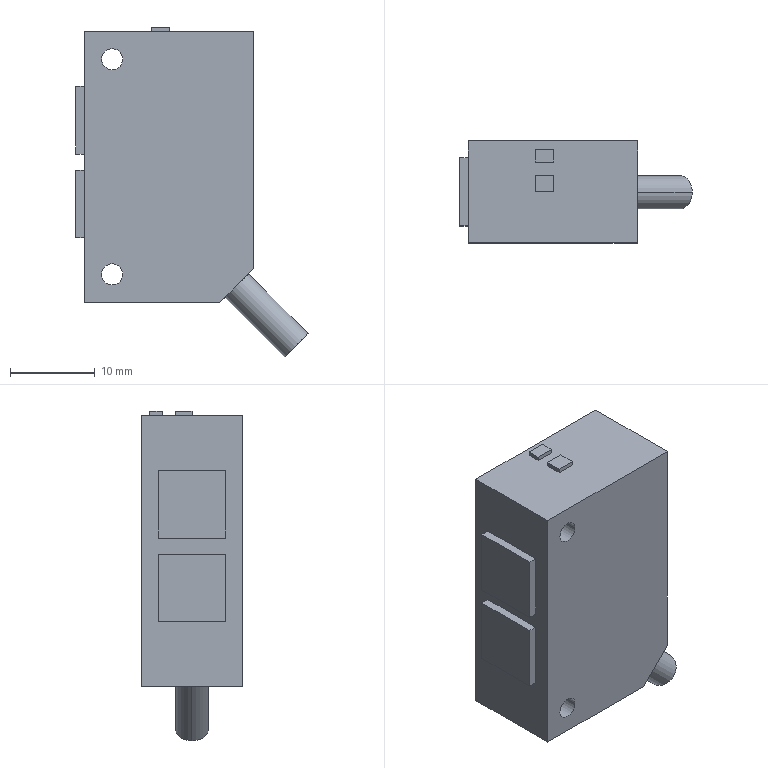Component | SolidWorks | Q20NRBanner-2 | 1 solid | 34 faces | box 27.45 x 12 x 38.95 mm | volume 7717 mm3 | plane 28 | cylinder 6 | commonest cylinder face diameters 2.5 x4 3.9 x2
build123d program:
from build123d import *

# Parameters (mm, degrees)
EXTRUDE1_DEPTH      = 6
EXTRUDE1_DEPTH_BACK = 6
SKETCH1_W           = 20
SKETCH1_H           = 32
M3_TAPPED_HOLE1_D   = 2.5
CHAMFER1_SIZE       = 4
SKETCH4_R           = 1.95
EXTRUDE2_DEPTH      = 10
SKETCH5_W           = 8
SKETCH5_H           = 8
EXTRUDE3_DEPTH      = 1
SKETCH12_W          = 2.2
SKETCH12_H          = 1.5
SKETCH12_H_2        = 1.92
EXTRUDE5_DEPTH      = 0.5


with BuildPart() as part:
    # Sketch1 → Extrude1 (new, two sides: drawn at the far end of the back side and taken through both)
    with BuildSketch(Plane.XY.offset(-EXTRUDE1_DEPTH_BACK)):
        with Locations((10, 16)):
            Rectangle(SKETCH1_W, SKETCH1_H)
    extrude(amount=EXTRUDE1_DEPTH + EXTRUDE1_DEPTH_BACK)

    # M3 Tapped Hole1 (through all)
    with Locations(Plane.XY.offset(6)):
        with Locations((3.3, 28.7), (3.3, 3.3)):
            Hole(M3_TAPPED_HOLE1_D / 2)

    # Chamfer1
    chamfer1_edges = [part.edges().sort_by_distance(p)[0] for p in [
        (20, 0, 0),
    ]]
    chamfer(chamfer1_edges, length=CHAMFER1_SIZE)

    # Sketch4 → Extrude2 (add)
    with BuildSketch(Plane(origin=(8, -8, 0), x_dir=(0, 0, -1), z_dir=(0.7071, -0.7071, 0))):
        with Locations(Location((0, 14.141, 0), (0, 0, 90))):
            Circle(SKETCH4_R)
    extrude(amount=EXTRUDE2_DEPTH)

    # Sketch5 → Extrude3 (add)
    with BuildSketch(Plane(origin=(0, 0, 0), x_dir=(0, 0, -1), z_dir=(1, 0, 0))):
        with Locations((0, 21.5)):
            Rectangle(SKETCH5_W, SKETCH5_H)
        with Locations((0, 11.6)):
            Rectangle(SKETCH5_W, SKETCH5_H)
    extrude(amount=-EXTRUDE3_DEPTH)

    # Sketch12 → Extrude5 (add)
    with BuildSketch(Plane(origin=(0, 32, 0), x_dir=(1, 0, 0), z_dir=(0, 1, 0))):
        with Locations((9, 4.25)):
            Rectangle(SKETCH12_W, SKETCH12_H)
        with Locations((9, 0.9598)):
            Rectangle(SKETCH12_W, SKETCH12_H_2)
    extrude(amount=EXTRUDE5_DEPTH)


solid = part.part

# Placed as in the assembly
solid = solid.moved(Location((-451.508, -99.092, 269.188), (90, 0, 0)))
STEP:
#1=CARTESIAN_POINT('',(-16.735,-3.901,10.453));
#2=VERTEX_POINT('',#1);
#3=CARTESIAN_POINT('',(-16.843,-3.901,10.344));
#4=VERTEX_POINT('',#3);
#5=CARTESIAN_POINT('',(-16.789,-3.901,10.398));
#6=DIRECTION('',(0.7071,0.,-0.7071));
#7=DIRECTION('',(0.7071,0.,0.7071));
#8=AXIS2_PLACEMENT_3D('',#5,#6,#7);
#9=CIRCLE('',#8,0.07677);
#10=EDGE_CURVE('',#2,#4,#9,.T.);
#11=ORIENTED_EDGE('',*,*,#10,.F.);
#12=CARTESIAN_POINT('',(-17.013,-3.901,10.731));
#13=VERTEX_POINT('',#12);
#14=CARTESIAN_POINT('',(-16.735,-3.901,10.453));
#15=DIRECTION('',(-0.7071,-0.,0.7071));
#16=VECTOR('',#15,39.37);
#17=LINE('',#14,#16);
#18=EDGE_CURVE('',#2,#13,#17,.T.);
#19=ORIENTED_EDGE('',*,*,#18,.T.);
#20=CARTESIAN_POINT('',(-17.122,-3.901,10.622));
#21=VERTEX_POINT('',#20);
#22=CARTESIAN_POINT('',(-17.067,-3.901,10.677));
#23=DIRECTION('',(0.7071,0.,-0.7071));
#24=DIRECTION('',(0.7071,0.,0.7071));
#25=AXIS2_PLACEMENT_3D('',#22,#23,#24);
#26=CIRCLE('',#25,0.07677);
#27=EDGE_CURVE('',#13,#21,#26,.T.);
#28=ORIENTED_EDGE('',*,*,#27,.T.);
#29=CARTESIAN_POINT('',(-16.843,-3.901,10.344));
#30=DIRECTION('',(-0.7071,-0.,0.7071));
#31=VECTOR('',#30,39.37);
#32=LINE('',#29,#31);
#33=EDGE_CURVE('',#4,#21,#32,.T.);
#34=ORIENTED_EDGE('',*,*,#33,.F.);
#35=EDGE_LOOP('',(#11,#19,#28,#34));
#36=FACE_OUTER_BOUND('',#35,.T.);
#37=CARTESIAN_POINT('',(-16.789,-3.901,10.398));
#38=DIRECTION('',(-0.7071,-0.,0.7071));
#39=DIRECTION('',(-0.7071,-0.,-0.7071));
#40=AXIS2_PLACEMENT_3D('',#37,#38,#39);
#41=CYLINDRICAL_SURFACE('',#40,0.07677);
#42=ADVANCED_FACE('',(#36),#41,.T.);
#43=CARTESIAN_POINT('',(-17.695,-3.665,11.728));
#44=VERTEX_POINT('',#43);
#45=CARTESIAN_POINT('',(-17.597,-3.665,11.728));
#46=VERTEX_POINT('',#45);
#47=CARTESIAN_POINT('',(-17.646,-3.665,11.728));
#48=DIRECTION('',(0.,-1.,0.));
#49=DIRECTION('',(1.,0.,0.));
#50=AXIS2_PLACEMENT_3D('',#47,#48,#49);
#51=CIRCLE('',#50,0.04921);
#52=EDGE_CURVE('',#44,#46,#51,.T.);
#53=ORIENTED_EDGE('',*,*,#52,.F.);
#54=CARTESIAN_POINT('',(-17.695,-4.137,11.728));
#55=VERTEX_POINT('',#54);
#56=CARTESIAN_POINT('',(-17.695,-4.137,11.728));
#57=DIRECTION('',(0.,-1.,0.));
#58=VECTOR('',#57,39.37);
#59=LINE('',#56,#58);
#60=EDGE_CURVE('',#44,#55,#59,.T.);
#61=ORIENTED_EDGE('',*,*,#60,.T.);
#62=CARTESIAN_POINT('',(-17.597,-4.137,11.728));
#63=VERTEX_POINT('',#62);
#64=CARTESIAN_POINT('',(-17.646,-4.137,11.728));
#65=DIRECTION('',(0.,-1.,0.));
#66=DIRECTION('',(1.,0.,0.));
#67=AXIS2_PLACEMENT_3D('',#64,#65,#66);
#68=CIRCLE('',#67,0.04921);
#69=EDGE_CURVE('',#55,#63,#68,.T.);
#70=ORIENTED_EDGE('',*,*,#69,.T.);
#71=CARTESIAN_POINT('',(-17.597,-4.137,11.728));
#72=DIRECTION('',(0.,-1.,0.));
#73=VECTOR('',#72,39.37);
#74=LINE('',#71,#73);
#75=EDGE_CURVE('',#46,#63,#74,.T.);
#76=ORIENTED_EDGE('',*,*,#75,.F.);
#77=EDGE_LOOP('',(#53,#61,#70,#76));
#78=FACE_OUTER_BOUND('',#77,.T.);
#79=CARTESIAN_POINT('',(-17.646,-4.137,11.728));
#80=DIRECTION('',(0.,-1.,0.));
#81=DIRECTION('',(1.,0.,0.));
#82=AXIS2_PLACEMENT_3D('',#79,#80,#81);
#83=CYLINDRICAL_SURFACE('',#82,0.04921);
#84=ADVANCED_FACE('',(#78),#83,.F.);
#85=CARTESIAN_POINT('',(-17.695,-3.665,10.728));
#86=VERTEX_POINT('',#85);
#87=CARTESIAN_POINT('',(-17.597,-3.665,10.728));
#88=VERTEX_POINT('',#87);
#89=CARTESIAN_POINT('',(-17.646,-3.665,10.728));
#90=DIRECTION('',(0.,-1.,0.));
#91=DIRECTION('',(1.,0.,0.));
#92=AXIS2_PLACEMENT_3D('',#89,#90,#91);
#93=CIRCLE('',#92,0.04921);
#94=EDGE_CURVE('',#86,#88,#93,.T.);
#95=ORIENTED_EDGE('',*,*,#94,.F.);
#96=CARTESIAN_POINT('',(-17.695,-4.137,10.728));
#97=VERTEX_POINT('',#96);
#98=CARTESIAN_POINT('',(-17.695,-4.137,10.728));
#99=DIRECTION('',(0.,-1.,0.));
#100=VECTOR('',#99,39.37);
#101=LINE('',#98,#100);
#102=EDGE_CURVE('',#86,#97,#101,.T.);
#103=ORIENTED_EDGE('',*,*,#102,.T.);
#104=CARTESIAN_POINT('',(-17.597,-4.137,10.728));
#105=VERTEX_POINT('',#104);
#106=CARTESIAN_POINT('',(-17.646,-4.137,10.728));
#107=DIRECTION('',(0.,-1.,0.));
#108=DIRECTION('',(1.,0.,0.));
#109=AXIS2_PLACEMENT_3D('',#106,#107,#108);
#110=CIRCLE('',#109,0.04921);
#111=EDGE_CURVE('',#97,#105,#110,.T.);
#112=ORIENTED_EDGE('',*,*,#111,.T.);
#113=CARTESIAN_POINT('',(-17.597,-4.137,10.728));
#114=DIRECTION('',(0.,-1.,0.));
#115=VECTOR('',#114,39.37);
#116=LINE('',#113,#115);
#117=EDGE_CURVE('',#88,#105,#116,.T.);
#118=ORIENTED_EDGE('',*,*,#117,.F.);
#119=EDGE_LOOP('',(#95,#103,#112,#118));
#120=FACE_OUTER_BOUND('',#119,.T.);
#121=CARTESIAN_POINT('',(-17.646,-4.137,10.728));
#122=DIRECTION('',(0.,-1.,0.));
#123=DIRECTION('',(1.,0.,0.));
#124=AXIS2_PLACEMENT_3D('',#121,#122,#123);
#125=CYLINDRICAL_SURFACE('',#124,0.04921);
#126=ADVANCED_FACE('',(#120),#125,.F.);
#127=CARTESIAN_POINT('',(-17.465,-3.763,11.858));
#128=VERTEX_POINT('',#127);
#129=CARTESIAN_POINT('',(-17.378,-3.763,11.858));
#130=VERTEX_POINT('',#129);
#131=CARTESIAN_POINT('',(-17.465,-3.763,11.858));
#132=DIRECTION('',(1.,0.,-0.));
#133=VECTOR('',#132,39.37);
#134=LINE('',#131,#133);
#135=EDGE_CURVE('',#128,#130,#134,.T.);
#136=ORIENTED_EDGE('',*,*,#135,.F.);
#137=CARTESIAN_POINT('',(-17.465,-3.704,11.858));
#138=VERTEX_POINT('',#137);
#139=CARTESIAN_POINT('',(-17.465,-3.704,11.858));
#140=DIRECTION('',(0.,-1.,0.));
#141=VECTOR('',#140,39.37);
#142=LINE('',#139,#141);
#143=EDGE_CURVE('',#138,#128,#142,.T.);
#144=ORIENTED_EDGE('',*,*,#143,.F.);
#145=CARTESIAN_POINT('',(-17.378,-3.704,11.858));
#146=VERTEX_POINT('',#145);
#147=CARTESIAN_POINT('',(-17.465,-3.704,11.858));
#148=DIRECTION('',(-1.,-0.,0.));
#149=VECTOR('',#148,39.37);
#150=LINE('',#147,#149);
#151=EDGE_CURVE('',#146,#138,#150,.T.);
#152=ORIENTED_EDGE('',*,*,#151,.F.);
#153=CARTESIAN_POINT('',(-17.378,-3.704,11.858));
#154=DIRECTION('',(-0.,1.,-0.));
#155=VECTOR('',#154,39.37);
#156=LINE('',#153,#155);
#157=EDGE_CURVE('',#130,#146,#156,.T.);
#158=ORIENTED_EDGE('',*,*,#157,.F.);
#159=EDGE_LOOP('',(#136,#144,#152,#158));
#160=FACE_BOUND('',#159,.T.);
#161=CARTESIAN_POINT('',(-17.776,-3.665,11.858));
#162=VERTEX_POINT('',#161);
#163=CARTESIAN_POINT('',(-17.776,-4.137,11.858));
#164=VERTEX_POINT('',#163);
#165=CARTESIAN_POINT('',(-17.776,-3.665,11.858));
#166=DIRECTION('',(0.,-1.,0.));
#167=VECTOR('',#166,39.37);
#168=LINE('',#165,#167);
#169=EDGE_CURVE('',#162,#164,#168,.T.);
#170=ORIENTED_EDGE('',*,*,#169,.T.);
#171=CARTESIAN_POINT('',(-16.988,-4.137,11.858));
#172=VERTEX_POINT('',#171);
#173=CARTESIAN_POINT('',(-17.776,-4.137,11.858));
#174=DIRECTION('',(-1.,-0.,0.));
#175=VECTOR('',#174,39.37);
#176=LINE('',#173,#175);
#177=EDGE_CURVE('',#172,#164,#176,.T.);
#178=ORIENTED_EDGE('',*,*,#177,.F.);
#179=CARTESIAN_POINT('',(-16.988,-3.665,11.858));
#180=VERTEX_POINT('',#179);
#181=CARTESIAN_POINT('',(-16.988,-3.665,11.858));
#182=DIRECTION('',(0.,-1.,0.));
#183=VECTOR('',#182,39.37);
#184=LINE('',#181,#183);
#185=EDGE_CURVE('',#180,#172,#184,.T.);
#186=ORIENTED_EDGE('',*,*,#185,.F.);
#187=CARTESIAN_POINT('',(-17.776,-3.665,11.858));
#188=DIRECTION('',(-1.,-0.,0.));
#189=VECTOR('',#188,39.37);
#190=LINE('',#187,#189);
#191=EDGE_CURVE('',#180,#162,#190,.T.);
#192=ORIENTED_EDGE('',*,*,#191,.T.);
#193=EDGE_LOOP('',(#170,#178,#186,#192));
#194=FACE_OUTER_BOUND('',#193,.T.);
#195=CARTESIAN_POINT('',(-17.465,-3.901,11.858));
#196=VERTEX_POINT('',#195);
#197=CARTESIAN_POINT('',(-17.378,-3.901,11.858));
#198=VERTEX_POINT('',#197);
#199=CARTESIAN_POINT('',(-17.465,-3.901,11.858));
#200=DIRECTION('',(1.,0.,-0.));
#201=VECTOR('',#200,39.37);
#202=LINE('',#199,#201);
#203=EDGE_CURVE('',#196,#198,#202,.T.);
#204=ORIENTED_EDGE('',*,*,#203,.F.);
#205=CARTESIAN_POINT('',(-17.465,-3.826,11.858));
#206=VERTEX_POINT('',#205);
#207=CARTESIAN_POINT('',(-17.465,-3.826,11.858));
#208=DIRECTION('',(0.,-1.,0.));
#209=VECTOR('',#208,39.37);
#210=LINE('',#207,#209);
#211=EDGE_CURVE('',#206,#196,#210,.T.);
#212=ORIENTED_EDGE('',*,*,#211,.F.);
#213=CARTESIAN_POINT('',(-17.378,-3.826,11.858));
#214=VERTEX_POINT('',#213);
#215=CARTESIAN_POINT('',(-17.465,-3.826,11.858));
#216=DIRECTION('',(-1.,-0.,0.));
#217=VECTOR('',#216,39.37);
#218=LINE('',#215,#217);
#219=EDGE_CURVE('',#214,#206,#218,.T.);
#220=ORIENTED_EDGE('',*,*,#219,.F.);
#221=CARTESIAN_POINT('',(-17.378,-3.826,11.858));
#222=DIRECTION('',(-0.,1.,-0.));
#223=VECTOR('',#222,39.37);
#224=LINE('',#221,#223);
#225=EDGE_CURVE('',#198,#214,#224,.T.);
#226=ORIENTED_EDGE('',*,*,#225,.F.);
#227=EDGE_LOOP('',(#204,#212,#220,#226));
#228=FACE_BOUND('',#227,.T.);
#229=CARTESIAN_POINT('',(-17.776,-3.665,11.858));
#230=DIRECTION('',(0.,0.,1.));
#231=DIRECTION('',(0.,-1.,0.));
#232=AXIS2_PLACEMENT_3D('',#229,#230,#231);
#233=PLANE('',#232);
#234=ADVANCED_FACE('',(#160,#194,#228),#233,.T.);
#235=CARTESIAN_POINT('',(-16.988,-3.665,10.755));
#236=VERTEX_POINT('',#235);
#237=CARTESIAN_POINT('',(-17.146,-3.665,10.598));
#238=VERTEX_POINT('',#237);
#239=CARTESIAN_POINT('',(-16.831,-3.665,10.913));
#240=DIRECTION('',(-0.7071,-0.,-0.7071));
#241=VECTOR('',#240,39.37);
#242=LINE('',#239,#241);
#243=EDGE_CURVE('',#236,#238,#242,.T.);
#244=ORIENTED_EDGE('',*,*,#243,.F.);
#245=CARTESIAN_POINT('',(-16.988,-4.137,10.755));
#246=VERTEX_POINT('',#245);
#247=CARTESIAN_POINT('',(-16.988,-3.665,10.755));
#248=DIRECTION('',(-0.,1.,-0.));
#249=VECTOR('',#248,39.37);
#250=LINE('',#247,#249);
#251=EDGE_CURVE('',#246,#236,#250,.T.);
#252=ORIENTED_EDGE('',*,*,#251,.F.);
#253=CARTESIAN_POINT('',(-17.146,-4.137,10.598));
#254=VERTEX_POINT('',#253);
#255=CARTESIAN_POINT('',(-17.146,-4.137,10.598));
#256=DIRECTION('',(0.7071,0.,0.7071));
#257=VECTOR('',#256,39.37);
#258=LINE('',#255,#257);
#259=EDGE_CURVE('',#254,#246,#258,.T.);
#260=ORIENTED_EDGE('',*,*,#259,.F.);
#261=CARTESIAN_POINT('',(-17.146,-3.665,10.598));
#262=DIRECTION('',(0.,-1.,0.));
#263=VECTOR('',#262,39.37);
#264=LINE('',#261,#263);
#265=EDGE_CURVE('',#238,#254,#264,.T.);
#266=ORIENTED_EDGE('',*,*,#265,.F.);
#267=EDGE_LOOP('',(#244,#252,#260,#266));
#268=FACE_OUTER_BOUND('',#267,.T.);
#269=CARTESIAN_POINT('',(-17.067,-3.901,10.677));
#270=DIRECTION('',(0.7071,0.,-0.7071));
#271=DIRECTION('',(0.7071,0.,0.7071));
#272=AXIS2_PLACEMENT_3D('',#269,#270,#271);
#273=CIRCLE('',#272,0.07677);
#274=EDGE_CURVE('',#21,#13,#273,.T.);
#275=ORIENTED_EDGE('',*,*,#274,.F.);
#276=ORIENTED_EDGE('',*,*,#27,.F.);
#277=EDGE_LOOP('',(#275,#276));
#278=FACE_BOUND('',#277,.T.);
#279=CARTESIAN_POINT('',(-17.146,-3.665,10.598));
#280=DIRECTION('',(-0.7071,-0.,0.7071));
#281=DIRECTION('',(-0.7071,-0.,-0.7071));
#282=AXIS2_PLACEMENT_3D('',#279,#280,#281);
#283=PLANE('',#282);
#284=ADVANCED_FACE('',(#268,#278),#283,.F.);
#285=CARTESIAN_POINT('',(-17.776,-4.059,11.212));
#286=VERTEX_POINT('',#285);
#287=CARTESIAN_POINT('',(-17.776,-4.059,10.897));
#288=VERTEX_POINT('',#287);
#289=CARTESIAN_POINT('',(-17.776,-4.059,11.212));
#290=DIRECTION('',(-0.,0.,-1.));
#291=VECTOR('',#290,39.37);
#292=LINE('',#289,#291);
#293=EDGE_CURVE('',#286,#288,#292,.T.);
#294=ORIENTED_EDGE('',*,*,#293,.T.);
#295=CARTESIAN_POINT('',(-17.776,-3.744,10.897));
#296=VERTEX_POINT('',#295);
#297=CARTESIAN_POINT('',(-17.776,-4.059,10.897));
#298=DIRECTION('',(-0.,1.,-0.));
#299=VECTOR('',#298,39.37);
#300=LINE('',#297,#299);
#301=EDGE_CURVE('',#288,#296,#300,.T.);
#302=ORIENTED_EDGE('',*,*,#301,.T.);
#303=CARTESIAN_POINT('',(-17.776,-3.744,11.212));
#304=VERTEX_POINT('',#303);
#305=CARTESIAN_POINT('',(-17.776,-3.744,11.212));
#306=DIRECTION('',(0.,-0.,1.));
#307=VECTOR('',#306,39.37);
#308=LINE('',#305,#307);
#309=EDGE_CURVE('',#296,#304,#308,.T.);
#310=ORIENTED_EDGE('',*,*,#309,.T.);
#311=CARTESIAN_POINT('',(-17.776,-4.059,11.212));
#312=DIRECTION('',(0.,-1.,-0.));
#313=VECTOR('',#312,39.37);
#314=LINE('',#311,#313);
#315=EDGE_CURVE('',#304,#286,#314,.T.);
#316=ORIENTED_EDGE('',*,*,#315,.T.);
#317=EDGE_LOOP('',(#294,#302,#310,#316));
#318=FACE_BOUND('',#317,.T.);
#319=CARTESIAN_POINT('',(-17.776,-4.059,11.602));
#320=VERTEX_POINT('',#319);
#321=CARTESIAN_POINT('',(-17.776,-4.059,11.287));
#322=VERTEX_POINT('',#321);
#323=CARTESIAN_POINT('',(-17.776,-4.059,11.602));
#324=DIRECTION('',(-0.,-0.,-1.));
#325=VECTOR('',#324,39.37);
#326=LINE('',#323,#325);
#327=EDGE_CURVE('',#320,#322,#326,.T.);
#328=ORIENTED_EDGE('',*,*,#327,.T.);
#329=CARTESIAN_POINT('',(-17.776,-3.744,11.287));
#330=VERTEX_POINT('',#329);
#331=CARTESIAN_POINT('',(-17.776,-4.059,11.287));
#332=DIRECTION('',(-0.,1.,-0.));
#333=VECTOR('',#332,39.37);
#334=LINE('',#331,#333);
#335=EDGE_CURVE('',#322,#330,#334,.T.);
#336=ORIENTED_EDGE('',*,*,#335,.T.);
#337=CARTESIAN_POINT('',(-17.776,-3.744,11.602));
#338=VERTEX_POINT('',#337);
#339=CARTESIAN_POINT('',(-17.776,-3.744,11.602));
#340=DIRECTION('',(0.,0.,1.));
#341=VECTOR('',#340,39.37);
#342=LINE('',#339,#341);
#343=EDGE_CURVE('',#330,#338,#342,.T.);
#344=ORIENTED_EDGE('',*,*,#343,.T.);
#345=CARTESIAN_POINT('',(-17.776,-4.059,11.602));
#346=DIRECTION('',(0.,-1.,0.));
#347=VECTOR('',#346,39.37);
#348=LINE('',#345,#347);
#349=EDGE_CURVE('',#338,#320,#348,.T.);
#350=ORIENTED_EDGE('',*,*,#349,.T.);
#351=EDGE_LOOP('',(#328,#336,#344,#350));
#352=FACE_BOUND('',#351,.T.);
#353=CARTESIAN_POINT('',(-17.776,-3.665,10.598));
#354=VERTEX_POINT('',#353);
#355=CARTESIAN_POINT('',(-17.776,-4.137,10.598));
#356=VERTEX_POINT('',#355);
#357=CARTESIAN_POINT('',(-17.776,-3.665,10.598));
#358=DIRECTION('',(0.,-1.,0.));
#359=VECTOR('',#358,39.37);
#360=LINE('',#357,#359);
#361=EDGE_CURVE('',#354,#356,#360,.T.);
#362=ORIENTED_EDGE('',*,*,#361,.T.);
#363=CARTESIAN_POINT('',(-17.776,-4.137,10.598));
#364=DIRECTION('',(-0.,-0.,-1.));
#365=VECTOR('',#364,39.37);
#366=LINE('',#363,#365);
#367=EDGE_CURVE('',#164,#356,#366,.T.);
#368=ORIENTED_EDGE('',*,*,#367,.F.);
#369=ORIENTED_EDGE('',*,*,#169,.F.);
#370=CARTESIAN_POINT('',(-17.776,-3.665,10.598));
#371=DIRECTION('',(-0.,-0.,-1.));
#372=VECTOR('',#371,39.37);
#373=LINE('',#370,#372);
#374=EDGE_CURVE('',#162,#354,#373,.T.);
#375=ORIENTED_EDGE('',*,*,#374,.T.);
#376=EDGE_LOOP('',(#362,#368,#369,#375));
#377=FACE_OUTER_BOUND('',#376,.T.);
#378=CARTESIAN_POINT('',(-17.776,-3.665,10.598));
#379=DIRECTION('',(-1.,-0.,0.));
#380=DIRECTION('',(0.,-1.,0.));
#381=AXIS2_PLACEMENT_3D('',#378,#379,#380);
#382=PLANE('',#381);
#383=ADVANCED_FACE('',(#318,#352,#377),#382,.T.);
#384=CARTESIAN_POINT('',(-16.988,-4.137,10.598));
#385=DIRECTION('',(0.,0.,1.));
#386=VECTOR('',#385,39.37);
#387=LINE('',#384,#386);
#388=EDGE_CURVE('',#246,#172,#387,.T.);
#389=ORIENTED_EDGE('',*,*,#388,.F.);
#390=ORIENTED_EDGE('',*,*,#251,.T.);
#391=CARTESIAN_POINT('',(-16.988,-3.665,10.598));
#392=DIRECTION('',(0.,0.,1.));
#393=VECTOR('',#392,39.37);
#394=LINE('',#391,#393);
#395=EDGE_CURVE('',#236,#180,#394,.T.);
#396=ORIENTED_EDGE('',*,*,#395,.T.);
#397=ORIENTED_EDGE('',*,*,#185,.T.);
#398=EDGE_LOOP('',(#389,#390,#396,#397));
#399=FACE_OUTER_BOUND('',#398,.T.);
#400=CARTESIAN_POINT('',(-16.988,-3.665,10.598));
#401=DIRECTION('',(1.,0.,-0.));
#402=DIRECTION('',(-0.,1.,-0.));
#403=AXIS2_PLACEMENT_3D('',#400,#401,#402);
#404=PLANE('',#403);
#405=ADVANCED_FACE('',(#399),#404,.T.);
#406=CARTESIAN_POINT('',(-17.776,-3.665,10.598));
#407=DIRECTION('',(1.,0.,-0.));
#408=VECTOR('',#407,39.37);
#409=LINE('',#406,#408);
#410=EDGE_CURVE('',#354,#238,#409,.T.);
#411=ORIENTED_EDGE('',*,*,#410,.T.);
#412=ORIENTED_EDGE('',*,*,#265,.T.);
#413=CARTESIAN_POINT('',(-17.776,-4.137,10.598));
#414=DIRECTION('',(1.,0.,-0.));
#415=VECTOR('',#414,39.37);
#416=LINE('',#413,#415);
#417=EDGE_CURVE('',#356,#254,#416,.T.);
#418=ORIENTED_EDGE('',*,*,#417,.F.);
#419=ORIENTED_EDGE('',*,*,#361,.F.);
#420=EDGE_LOOP('',(#411,#412,#418,#419));
#421=FACE_OUTER_BOUND('',#420,.T.);
#422=CARTESIAN_POINT('',(-17.776,-3.665,10.598));
#423=DIRECTION('',(-0.,-0.,-1.));
#424=DIRECTION('',(-0.,1.,-0.));
#425=AXIS2_PLACEMENT_3D('',#422,#423,#424);
#426=PLANE('',#425);
#427=ADVANCED_FACE('',(#421),#426,.T.);
#428=CARTESIAN_POINT('',(-17.646,-3.665,11.728));
#429=DIRECTION('',(0.,-1.,0.));
#430=DIRECTION('',(1.,0.,0.));
#431=AXIS2_PLACEMENT_3D('',#428,#429,#430);
#432=CIRCLE('',#431,0.04921);
#433=EDGE_CURVE('',#46,#44,#432,.T.);
#434=ORIENTED_EDGE('',*,*,#433,.T.);
#435=ORIENTED_EDGE('',*,*,#52,.T.);
#436=EDGE_LOOP('',(#434,#435));
#437=FACE_BOUND('',#436,.T.);
#438=CARTESIAN_POINT('',(-17.646,-3.665,10.728));
#439=DIRECTION('',(0.,-1.,0.));
#440=DIRECTION('',(1.,0.,0.));
#441=AXIS2_PLACEMENT_3D('',#438,#439,#440);
#442=CIRCLE('',#441,0.04921);
#443=EDGE_CURVE('',#88,#86,#442,.T.);
#444=ORIENTED_EDGE('',*,*,#443,.T.);
#445=ORIENTED_EDGE('',*,*,#94,.T.);
#446=EDGE_LOOP('',(#444,#445));
#447=FACE_BOUND('',#446,.T.);
#448=ORIENTED_EDGE('',*,*,#395,.F.);
#449=ORIENTED_EDGE('',*,*,#243,.T.);
#450=ORIENTED_EDGE('',*,*,#410,.F.);
#451=ORIENTED_EDGE('',*,*,#374,.F.);
#452=ORIENTED_EDGE('',*,*,#191,.F.);
#453=EDGE_LOOP('',(#448,#449,#450,#451,#452));
#454=FACE_OUTER_BOUND('',#453,.T.);
#455=CARTESIAN_POINT('',(-17.776,-3.665,11.858));
#456=DIRECTION('',(-0.,1.,-0.));
#457=DIRECTION('',(-1.,-0.,0.));
#458=AXIS2_PLACEMENT_3D('',#455,#456,#457);
#459=PLANE('',#458);
#460=ADVANCED_FACE('',(#437,#447,#454),#459,.T.);
#461=CARTESIAN_POINT('',(-17.646,-4.137,11.728));
#462=DIRECTION('',(0.,-1.,0.));
#463=DIRECTION('',(1.,0.,0.));
#464=AXIS2_PLACEMENT_3D('',#461,#462,#463);
#465=CIRCLE('',#464,0.04921);
#466=EDGE_CURVE('',#63,#55,#465,.T.);
#467=ORIENTED_EDGE('',*,*,#466,.F.);
#468=ORIENTED_EDGE('',*,*,#69,.F.);
#469=EDGE_LOOP('',(#467,#468));
#470=FACE_BOUND('',#469,.T.);
#471=CARTESIAN_POINT('',(-17.646,-4.137,10.728));
#472=DIRECTION('',(0.,-1.,0.));
#473=DIRECTION('',(1.,0.,0.));
#474=AXIS2_PLACEMENT_3D('',#471,#472,#473);
#475=CIRCLE('',#474,0.04921);
#476=EDGE_CURVE('',#105,#97,#475,.T.);
#477=ORIENTED_EDGE('',*,*,#476,.F.);
#478=ORIENTED_EDGE('',*,*,#111,.F.);
#479=EDGE_LOOP('',(#477,#478));
#480=FACE_BOUND('',#479,.T.);
#481=ORIENTED_EDGE('',*,*,#417,.T.);
#482=ORIENTED_EDGE('',*,*,#259,.T.);
#483=ORIENTED_EDGE('',*,*,#388,.T.);
#484=ORIENTED_EDGE('',*,*,#177,.T.);
#485=ORIENTED_EDGE('',*,*,#367,.T.);
#486=EDGE_LOOP('',(#481,#482,#483,#484,#485));
#487=FACE_OUTER_BOUND('',#486,.T.);
#488=CARTESIAN_POINT('',(-17.776,-4.137,11.858));
#489=DIRECTION('',(-0.,1.,-0.));
#490=DIRECTION('',(-1.,-0.,0.));
#491=AXIS2_PLACEMENT_3D('',#488,#489,#490);
#492=PLANE('',#491);
#493=ADVANCED_FACE('',(#470,#480,#487),#492,.F.);
#494=ORIENTED_EDGE('',*,*,#102,.F.);
#495=ORIENTED_EDGE('',*,*,#443,.F.);
#496=ORIENTED_EDGE('',*,*,#117,.T.);
#497=ORIENTED_EDGE('',*,*,#476,.T.);
#498=EDGE_LOOP('',(#494,#495,#496,#497));
#499=FACE_OUTER_BOUND('',#498,.T.);
#500=CARTESIAN_POINT('',(-17.646,-4.137,10.728));
#501=DIRECTION('',(0.,-1.,0.));
#502=DIRECTION('',(1.,0.,0.));
#503=AXIS2_PLACEMENT_3D('',#500,#501,#502);
#504=CYLINDRICAL_SURFACE('',#503,0.04921);
#505=ADVANCED_FACE('',(#499),#504,.F.);
#506=ORIENTED_EDGE('',*,*,#60,.F.);
#507=ORIENTED_EDGE('',*,*,#433,.F.);
#508=ORIENTED_EDGE('',*,*,#75,.T.);
#509=ORIENTED_EDGE('',*,*,#466,.T.);
#510=EDGE_LOOP('',(#506,#507,#508,#509));
#511=FACE_OUTER_BOUND('',#510,.T.);
#512=CARTESIAN_POINT('',(-17.646,-4.137,11.728));
#513=DIRECTION('',(0.,-1.,0.));
#514=DIRECTION('',(1.,0.,0.));
#515=AXIS2_PLACEMENT_3D('',#512,#513,#514);
#516=CYLINDRICAL_SURFACE('',#515,0.04921);
#517=ADVANCED_FACE('',(#511),#516,.F.);
#518=ORIENTED_EDGE('',*,*,#18,.F.);
#519=CARTESIAN_POINT('',(-16.789,-3.901,10.398));
#520=DIRECTION('',(0.7071,0.,-0.7071));
#521=DIRECTION('',(0.7071,0.,0.7071));
#522=AXIS2_PLACEMENT_3D('',#519,#520,#521);
#523=CIRCLE('',#522,0.07677);
#524=EDGE_CURVE('',#4,#2,#523,.T.);
#525=ORIENTED_EDGE('',*,*,#524,.F.);
#526=ORIENTED_EDGE('',*,*,#33,.T.);
#527=ORIENTED_EDGE('',*,*,#274,.T.);
#528=EDGE_LOOP('',(#518,#525,#526,#527));
#529=FACE_OUTER_BOUND('',#528,.T.);
#530=CARTESIAN_POINT('',(-16.789,-3.901,10.398));
#531=DIRECTION('',(-0.7071,-0.,0.7071));
#532=DIRECTION('',(-0.7071,-0.,-0.7071));
#533=AXIS2_PLACEMENT_3D('',#530,#531,#532);
#534=CYLINDRICAL_SURFACE('',#533,0.07677);
#535=ADVANCED_FACE('',(#529),#534,.T.);
#536=ORIENTED_EDGE('',*,*,#524,.T.);
#537=ORIENTED_EDGE('',*,*,#10,.T.);
#538=EDGE_LOOP('',(#536,#537));
#539=FACE_OUTER_BOUND('',#538,.T.);
#540=CARTESIAN_POINT('',(-16.789,-3.901,10.398));
#541=DIRECTION('',(0.7071,0.,-0.7071));
#542=DIRECTION('',(0.7071,0.,0.7071));
#543=AXIS2_PLACEMENT_3D('',#540,#541,#542);
#544=PLANE('',#543);
#545=ADVANCED_FACE('',(#539),#544,.T.);
#546=ORIENTED_EDGE('',*,*,#327,.F.);
#547=CARTESIAN_POINT('',(-17.815,-4.059,11.602));
#548=VERTEX_POINT('',#547);
#549=CARTESIAN_POINT('',(-17.815,-4.059,11.602));
#550=DIRECTION('',(1.,0.,-0.));
#551=VECTOR('',#550,39.37);
#552=LINE('',#549,#551);
#553=EDGE_CURVE('',#548,#320,#552,.T.);
#554=ORIENTED_EDGE('',*,*,#553,.F.);
#555=CARTESIAN_POINT('',(-17.815,-4.059,11.287));
#556=VERTEX_POINT('',#555);
#557=CARTESIAN_POINT('',(-17.815,-4.059,11.602));
#558=DIRECTION('',(-0.,-0.,-1.));
#559=VECTOR('',#558,39.37);
#560=LINE('',#557,#559);
#561=EDGE_CURVE('',#548,#556,#560,.T.);
#562=ORIENTED_EDGE('',*,*,#561,.T.);
#563=CARTESIAN_POINT('',(-17.815,-4.059,11.287));
#564=DIRECTION('',(1.,0.,-0.));
#565=VECTOR('',#564,39.37);
#566=LINE('',#563,#565);
#567=EDGE_CURVE('',#556,#322,#566,.T.);
#568=ORIENTED_EDGE('',*,*,#567,.T.);
#569=EDGE_LOOP('',(#546,#554,#562,#568));
#570=FACE_OUTER_BOUND('',#569,.T.);
#571=CARTESIAN_POINT('',(-17.815,-4.059,11.602));
#572=DIRECTION('',(0.,-1.,0.));
#573=DIRECTION('',(1.,0.,-0.));
#574=AXIS2_PLACEMENT_3D('',#571,#572,#573);
#575=PLANE('',#574);
#576=ADVANCED_FACE('',(#570),#575,.T.);
#577=ORIENTED_EDGE('',*,*,#349,.F.);
#578=CARTESIAN_POINT('',(-17.815,-3.744,11.602));
#579=VERTEX_POINT('',#578);
#580=CARTESIAN_POINT('',(-17.815,-3.744,11.602));
#581=DIRECTION('',(1.,0.,-0.));
#582=VECTOR('',#581,39.37);
#583=LINE('',#580,#582);
#584=EDGE_CURVE('',#579,#338,#583,.T.);
#585=ORIENTED_EDGE('',*,*,#584,.F.);
#586=CARTESIAN_POINT('',(-17.815,-4.059,11.602));
#587=DIRECTION('',(0.,-1.,0.));
#588=VECTOR('',#587,39.37);
#589=LINE('',#586,#588);
#590=EDGE_CURVE('',#579,#548,#589,.T.);
#591=ORIENTED_EDGE('',*,*,#590,.T.);
#592=ORIENTED_EDGE('',*,*,#553,.T.);
#593=EDGE_LOOP('',(#577,#585,#591,#592));
#594=FACE_OUTER_BOUND('',#593,.T.);
#595=CARTESIAN_POINT('',(-17.815,-4.059,11.602));
#596=DIRECTION('',(0.,0.,1.));
#597=DIRECTION('',(0.,-1.,0.));
#598=AXIS2_PLACEMENT_3D('',#595,#596,#597);
#599=PLANE('',#598);
#600=ADVANCED_FACE('',(#594),#599,.T.);
#601=ORIENTED_EDGE('',*,*,#343,.F.);
#602=CARTESIAN_POINT('',(-17.815,-3.744,11.287));
#603=VERTEX_POINT('',#602);
#604=CARTESIAN_POINT('',(-17.815,-3.744,11.287));
#605=DIRECTION('',(1.,0.,-0.));
#606=VECTOR('',#605,39.37);
#607=LINE('',#604,#606);
#608=EDGE_CURVE('',#603,#330,#607,.T.);
#609=ORIENTED_EDGE('',*,*,#608,.F.);
#610=CARTESIAN_POINT('',(-17.815,-3.744,11.602));
#611=DIRECTION('',(0.,0.,1.));
#612=VECTOR('',#611,39.37);
#613=LINE('',#610,#612);
#614=EDGE_CURVE('',#603,#579,#613,.T.);
#615=ORIENTED_EDGE('',*,*,#614,.T.);
#616=ORIENTED_EDGE('',*,*,#584,.T.);
#617=EDGE_LOOP('',(#601,#609,#615,#616));
#618=FACE_OUTER_BOUND('',#617,.T.);
#619=CARTESIAN_POINT('',(-17.815,-3.744,11.602));
#620=DIRECTION('',(-0.,1.,-0.));
#621=DIRECTION('',(-1.,-0.,0.));
#622=AXIS2_PLACEMENT_3D('',#619,#620,#621);
#623=PLANE('',#622);
#624=ADVANCED_FACE('',(#618),#623,.T.);
#625=ORIENTED_EDGE('',*,*,#335,.F.);
#626=ORIENTED_EDGE('',*,*,#567,.F.);
#627=CARTESIAN_POINT('',(-17.815,-4.059,11.287));
#628=DIRECTION('',(-0.,1.,-0.));
#629=VECTOR('',#628,39.37);
#630=LINE('',#627,#629);
#631=EDGE_CURVE('',#556,#603,#630,.T.);
#632=ORIENTED_EDGE('',*,*,#631,.T.);
#633=ORIENTED_EDGE('',*,*,#608,.T.);
#634=EDGE_LOOP('',(#625,#626,#632,#633));
#635=FACE_OUTER_BOUND('',#634,.T.);
#636=CARTESIAN_POINT('',(-17.815,-4.059,11.287));
#637=DIRECTION('',(-0.,-0.,-1.));
#638=DIRECTION('',(-0.,1.,-0.));
#639=AXIS2_PLACEMENT_3D('',#636,#637,#638);
#640=PLANE('',#639);
#641=ADVANCED_FACE('',(#635),#640,.T.);
#642=ORIENTED_EDGE('',*,*,#561,.F.);
#643=ORIENTED_EDGE('',*,*,#590,.F.);
#644=ORIENTED_EDGE('',*,*,#614,.F.);
#645=ORIENTED_EDGE('',*,*,#631,.F.);
#646=EDGE_LOOP('',(#642,#643,#644,#645));
#647=FACE_OUTER_BOUND('',#646,.T.);
#648=CARTESIAN_POINT('',(-17.815,-4.059,11.287));
#649=DIRECTION('',(1.,0.,-0.));
#650=DIRECTION('',(-0.,1.,-0.));
#651=AXIS2_PLACEMENT_3D('',#648,#649,#650);
#652=PLANE('',#651);
#653=ADVANCED_FACE('',(#647),#652,.F.);
#654=ORIENTED_EDGE('',*,*,#293,.F.);
#655=CARTESIAN_POINT('',(-17.815,-4.059,11.212));
#656=VERTEX_POINT('',#655);
#657=CARTESIAN_POINT('',(-17.815,-4.059,11.212));
#658=DIRECTION('',(1.,0.,-0.));
#659=VECTOR('',#658,39.37);
#660=LINE('',#657,#659);
#661=EDGE_CURVE('',#656,#286,#660,.T.);
#662=ORIENTED_EDGE('',*,*,#661,.F.);
#663=CARTESIAN_POINT('',(-17.815,-4.059,10.897));
#664=VERTEX_POINT('',#663);
#665=CARTESIAN_POINT('',(-17.815,-4.059,11.212));
#666=DIRECTION('',(-0.,0.,-1.));
#667=VECTOR('',#666,39.37);
#668=LINE('',#665,#667);
#669=EDGE_CURVE('',#656,#664,#668,.T.);
#670=ORIENTED_EDGE('',*,*,#669,.T.);
#671=CARTESIAN_POINT('',(-17.815,-4.059,10.897));
#672=DIRECTION('',(1.,0.,-0.));
#673=VECTOR('',#672,39.37);
#674=LINE('',#671,#673);
#675=EDGE_CURVE('',#664,#288,#674,.T.);
#676=ORIENTED_EDGE('',*,*,#675,.T.);
#677=EDGE_LOOP('',(#654,#662,#670,#676));
#678=FACE_OUTER_BOUND('',#677,.T.);
#679=CARTESIAN_POINT('',(-17.815,-4.059,11.212));
#680=DIRECTION('',(0.,-1.,-0.));
#681=DIRECTION('',(-0.,0.,-1.));
#682=AXIS2_PLACEMENT_3D('',#679,#680,#681);
#683=PLANE('',#682);
#684=ADVANCED_FACE('',(#678),#683,.T.);
#685=ORIENTED_EDGE('',*,*,#315,.F.);
#686=CARTESIAN_POINT('',(-17.815,-3.744,11.212));
#687=VERTEX_POINT('',#686);
#688=CARTESIAN_POINT('',(-17.815,-3.744,11.212));
#689=DIRECTION('',(1.,0.,-0.));
#690=VECTOR('',#689,39.37);
#691=LINE('',#688,#690);
#692=EDGE_CURVE('',#687,#304,#691,.T.);
#693=ORIENTED_EDGE('',*,*,#692,.F.);
#694=CARTESIAN_POINT('',(-17.815,-4.059,11.212));
#695=DIRECTION('',(0.,-1.,-0.));
#696=VECTOR('',#695,39.37);
#697=LINE('',#694,#696);
#698=EDGE_CURVE('',#687,#656,#697,.T.);
#699=ORIENTED_EDGE('',*,*,#698,.T.);
#700=ORIENTED_EDGE('',*,*,#661,.T.);
#701=EDGE_LOOP('',(#685,#693,#699,#700));
#702=FACE_OUTER_BOUND('',#701,.T.);
#703=CARTESIAN_POINT('',(-17.815,-4.059,11.212));
#704=DIRECTION('',(0.,-0.,1.));
#705=DIRECTION('',(0.,-1.,-0.));
#706=AXIS2_PLACEMENT_3D('',#703,#704,#705);
#707=PLANE('',#706);
#708=ADVANCED_FACE('',(#702),#707,.T.);
#709=ORIENTED_EDGE('',*,*,#309,.F.);
#710=CARTESIAN_POINT('',(-17.815,-3.744,10.897));
#711=VERTEX_POINT('',#710);
#712=CARTESIAN_POINT('',(-17.815,-3.744,10.897));
#713=DIRECTION('',(1.,0.,-0.));
#714=VECTOR('',#713,39.37);
#715=LINE('',#712,#714);
#716=EDGE_CURVE('',#711,#296,#715,.T.);
#717=ORIENTED_EDGE('',*,*,#716,.F.);
#718=CARTESIAN_POINT('',(-17.815,-3.744,11.212));
#719=DIRECTION('',(0.,-0.,1.));
#720=VECTOR('',#719,39.37);
#721=LINE('',#718,#720);
#722=EDGE_CURVE('',#711,#687,#721,.T.);
#723=ORIENTED_EDGE('',*,*,#722,.T.);
#724=ORIENTED_EDGE('',*,*,#692,.T.);
#725=EDGE_LOOP('',(#709,#717,#723,#724));
#726=FACE_OUTER_BOUND('',#725,.T.);
#727=CARTESIAN_POINT('',(-17.815,-3.744,11.212));
#728=DIRECTION('',(-0.,1.,0.));
#729=DIRECTION('',(0.,-0.,1.));
#730=AXIS2_PLACEMENT_3D('',#727,#728,#729);
#731=PLANE('',#730);
#732=ADVANCED_FACE('',(#726),#731,.T.);
#733=ORIENTED_EDGE('',*,*,#301,.F.);
#734=ORIENTED_EDGE('',*,*,#675,.F.);
#735=CARTESIAN_POINT('',(-17.815,-4.059,10.897));
#736=DIRECTION('',(-0.,1.,-0.));
#737=VECTOR('',#736,39.37);
#738=LINE('',#735,#737);
#739=EDGE_CURVE('',#664,#711,#738,.T.);
#740=ORIENTED_EDGE('',*,*,#739,.T.);
#741=ORIENTED_EDGE('',*,*,#716,.T.);
#742=EDGE_LOOP('',(#733,#734,#740,#741));
#743=FACE_OUTER_BOUND('',#742,.T.);
#744=CARTESIAN_POINT('',(-17.815,-4.059,10.897));
#745=DIRECTION('',(-0.,-0.,-1.));
#746=DIRECTION('',(-0.,1.,-0.));
#747=AXIS2_PLACEMENT_3D('',#744,#745,#746);
#748=PLANE('',#747);
#749=ADVANCED_FACE('',(#743),#748,.T.);
#750=ORIENTED_EDGE('',*,*,#669,.F.);
#751=ORIENTED_EDGE('',*,*,#698,.F.);
#752=ORIENTED_EDGE('',*,*,#722,.F.);
#753=ORIENTED_EDGE('',*,*,#739,.F.);
#754=EDGE_LOOP('',(#750,#751,#752,#753));
#755=FACE_OUTER_BOUND('',#754,.T.);
#756=CARTESIAN_POINT('',(-17.815,-4.059,11.212));
#757=DIRECTION('',(1.,0.,-0.));
#758=DIRECTION('',(-0.,1.,-0.));
#759=AXIS2_PLACEMENT_3D('',#756,#757,#758);
#760=PLANE('',#759);
#761=ADVANCED_FACE('',(#755),#760,.F.);
#762=ORIENTED_EDGE('',*,*,#143,.T.);
#763=CARTESIAN_POINT('',(-17.465,-3.763,11.877));
#764=VERTEX_POINT('',#763);
#765=CARTESIAN_POINT('',(-17.465,-3.763,11.877));
#766=DIRECTION('',(-0.,-0.,-1.));
#767=VECTOR('',#766,39.37);
#768=LINE('',#765,#767);
#769=EDGE_CURVE('',#764,#128,#768,.T.);
#770=ORIENTED_EDGE('',*,*,#769,.F.);
#771=CARTESIAN_POINT('',(-17.465,-3.704,11.877));
#772=VERTEX_POINT('',#771);
#773=CARTESIAN_POINT('',(-17.465,-3.704,11.877));
#774=DIRECTION('',(0.,-1.,0.));
#775=VECTOR('',#774,39.37);
#776=LINE('',#773,#775);
#777=EDGE_CURVE('',#772,#764,#776,.T.);
#778=ORIENTED_EDGE('',*,*,#777,.F.);
#779=CARTESIAN_POINT('',(-17.465,-3.704,11.877));
#780=DIRECTION('',(-0.,-0.,-1.));
#781=VECTOR('',#780,39.37);
#782=LINE('',#779,#781);
#783=EDGE_CURVE('',#772,#138,#782,.T.);
#784=ORIENTED_EDGE('',*,*,#783,.T.);
#785=EDGE_LOOP('',(#762,#770,#778,#784));
#786=FACE_OUTER_BOUND('',#785,.T.);
#787=CARTESIAN_POINT('',(-17.465,-3.704,11.877));
#788=DIRECTION('',(1.,0.,-0.));
#789=DIRECTION('',(-0.,1.,-0.));
#790=AXIS2_PLACEMENT_3D('',#787,#788,#789);
#791=PLANE('',#790);
#792=ADVANCED_FACE('',(#786),#791,.F.);
#793=ORIENTED_EDGE('',*,*,#135,.T.);
#794=CARTESIAN_POINT('',(-17.378,-3.763,11.877));
#795=VERTEX_POINT('',#794);
#796=CARTESIAN_POINT('',(-17.378,-3.763,11.877));
#797=DIRECTION('',(-0.,-0.,-1.));
#798=VECTOR('',#797,39.37);
#799=LINE('',#796,#798);
#800=EDGE_CURVE('',#795,#130,#799,.T.);
#801=ORIENTED_EDGE('',*,*,#800,.F.);
#802=CARTESIAN_POINT('',(-17.465,-3.763,11.877));
#803=DIRECTION('',(1.,0.,-0.));
#804=VECTOR('',#803,39.37);
#805=LINE('',#802,#804);
#806=EDGE_CURVE('',#764,#795,#805,.T.);
#807=ORIENTED_EDGE('',*,*,#806,.F.);
#808=ORIENTED_EDGE('',*,*,#769,.T.);
#809=EDGE_LOOP('',(#793,#801,#807,#808));
#810=FACE_OUTER_BOUND('',#809,.T.);
#811=CARTESIAN_POINT('',(-17.465,-3.763,11.877));
#812=DIRECTION('',(-0.,1.,-0.));
#813=DIRECTION('',(-1.,-0.,0.));
#814=AXIS2_PLACEMENT_3D('',#811,#812,#813);
#815=PLANE('',#814);
#816=ADVANCED_FACE('',(#810),#815,.F.);
#817=ORIENTED_EDGE('',*,*,#157,.T.);
#818=CARTESIAN_POINT('',(-17.378,-3.704,11.877));
#819=VERTEX_POINT('',#818);
#820=CARTESIAN_POINT('',(-17.378,-3.704,11.877));
#821=DIRECTION('',(-0.,-0.,-1.));
#822=VECTOR('',#821,39.37);
#823=LINE('',#820,#822);
#824=EDGE_CURVE('',#819,#146,#823,.T.);
#825=ORIENTED_EDGE('',*,*,#824,.F.);
#826=CARTESIAN_POINT('',(-17.378,-3.704,11.877));
#827=DIRECTION('',(-0.,1.,-0.));
#828=VECTOR('',#827,39.37);
#829=LINE('',#826,#828);
#830=EDGE_CURVE('',#795,#819,#829,.T.);
#831=ORIENTED_EDGE('',*,*,#830,.F.);
#832=ORIENTED_EDGE('',*,*,#800,.T.);
#833=EDGE_LOOP('',(#817,#825,#831,#832));
#834=FACE_OUTER_BOUND('',#833,.T.);
#835=CARTESIAN_POINT('',(-17.378,-3.704,11.877));
#836=DIRECTION('',(-1.,-0.,0.));
#837=DIRECTION('',(0.,-1.,0.));
#838=AXIS2_PLACEMENT_3D('',#835,#836,#837);
#839=PLANE('',#838);
#840=ADVANCED_FACE('',(#834),#839,.F.);
#841=ORIENTED_EDGE('',*,*,#151,.T.);
#842=ORIENTED_EDGE('',*,*,#783,.F.);
#843=CARTESIAN_POINT('',(-17.465,-3.704,11.877));
#844=DIRECTION('',(-1.,-0.,0.));
#845=VECTOR('',#844,39.37);
#846=LINE('',#843,#845);
#847=EDGE_CURVE('',#819,#772,#846,.T.);
#848=ORIENTED_EDGE('',*,*,#847,.F.);
#849=ORIENTED_EDGE('',*,*,#824,.T.);
#850=EDGE_LOOP('',(#841,#842,#848,#849));
#851=FACE_OUTER_BOUND('',#850,.T.);
#852=CARTESIAN_POINT('',(-17.465,-3.704,11.877));
#853=DIRECTION('',(0.,-1.,0.));
#854=DIRECTION('',(1.,0.,-0.));
#855=AXIS2_PLACEMENT_3D('',#852,#853,#854);
#856=PLANE('',#855);
#857=ADVANCED_FACE('',(#851),#856,.F.);
#858=ORIENTED_EDGE('',*,*,#777,.T.);
#859=ORIENTED_EDGE('',*,*,#806,.T.);
#860=ORIENTED_EDGE('',*,*,#830,.T.);
#861=ORIENTED_EDGE('',*,*,#847,.T.);
#862=EDGE_LOOP('',(#858,#859,#860,#861));
#863=FACE_OUTER_BOUND('',#862,.T.);
#864=CARTESIAN_POINT('',(-17.465,-3.763,11.877));
#865=DIRECTION('',(0.,0.,1.));
#866=DIRECTION('',(0.,-1.,0.));
#867=AXIS2_PLACEMENT_3D('',#864,#865,#866);
#868=PLANE('',#867);
#869=ADVANCED_FACE('',(#863),#868,.T.);
#870=ORIENTED_EDGE('',*,*,#211,.T.);
#871=CARTESIAN_POINT('',(-17.465,-3.901,11.877));
#872=VERTEX_POINT('',#871);
#873=CARTESIAN_POINT('',(-17.465,-3.901,11.877));
#874=DIRECTION('',(-0.,-0.,-1.));
#875=VECTOR('',#874,39.37);
#876=LINE('',#873,#875);
#877=EDGE_CURVE('',#872,#196,#876,.T.);
#878=ORIENTED_EDGE('',*,*,#877,.F.);
#879=CARTESIAN_POINT('',(-17.465,-3.826,11.877));
#880=VERTEX_POINT('',#879);
#881=CARTESIAN_POINT('',(-17.465,-3.826,11.877));
#882=DIRECTION('',(0.,-1.,0.));
#883=VECTOR('',#882,39.37);
#884=LINE('',#881,#883);
#885=EDGE_CURVE('',#880,#872,#884,.T.);
#886=ORIENTED_EDGE('',*,*,#885,.F.);
#887=CARTESIAN_POINT('',(-17.465,-3.826,11.877));
#888=DIRECTION('',(-0.,-0.,-1.));
#889=VECTOR('',#888,39.37);
#890=LINE('',#887,#889);
#891=EDGE_CURVE('',#880,#206,#890,.T.);
#892=ORIENTED_EDGE('',*,*,#891,.T.);
#893=EDGE_LOOP('',(#870,#878,#886,#892));
#894=FACE_OUTER_BOUND('',#893,.T.);
#895=CARTESIAN_POINT('',(-17.465,-3.826,11.877));
#896=DIRECTION('',(1.,0.,-0.));
#897=DIRECTION('',(-0.,1.,-0.));
#898=AXIS2_PLACEMENT_3D('',#895,#896,#897);
#899=PLANE('',#898);
#900=ADVANCED_FACE('',(#894),#899,.F.);
#901=ORIENTED_EDGE('',*,*,#203,.T.);
#902=CARTESIAN_POINT('',(-17.378,-3.901,11.877));
#903=VERTEX_POINT('',#902);
#904=CARTESIAN_POINT('',(-17.378,-3.901,11.877));
#905=DIRECTION('',(-0.,-0.,-1.));
#906=VECTOR('',#905,39.37);
#907=LINE('',#904,#906);
#908=EDGE_CURVE('',#903,#198,#907,.T.);
#909=ORIENTED_EDGE('',*,*,#908,.F.);
#910=CARTESIAN_POINT('',(-17.465,-3.901,11.877));
#911=DIRECTION('',(1.,0.,-0.));
#912=VECTOR('',#911,39.37);
#913=LINE('',#910,#912);
#914=EDGE_CURVE('',#872,#903,#913,.T.);
#915=ORIENTED_EDGE('',*,*,#914,.F.);
#916=ORIENTED_EDGE('',*,*,#877,.T.);
#917=EDGE_LOOP('',(#901,#909,#915,#916));
#918=FACE_OUTER_BOUND('',#917,.T.);
#919=CARTESIAN_POINT('',(-17.465,-3.901,11.877));
#920=DIRECTION('',(-0.,1.,-0.));
#921=DIRECTION('',(-1.,-0.,0.));
#922=AXIS2_PLACEMENT_3D('',#919,#920,#921);
#923=PLANE('',#922);
#924=ADVANCED_FACE('',(#918),#923,.F.);
#925=ORIENTED_EDGE('',*,*,#225,.T.);
#926=CARTESIAN_POINT('',(-17.378,-3.826,11.877));
#927=VERTEX_POINT('',#926);
#928=CARTESIAN_POINT('',(-17.378,-3.826,11.877));
#929=DIRECTION('',(-0.,-0.,-1.));
#930=VECTOR('',#929,39.37);
#931=LINE('',#928,#930);
#932=EDGE_CURVE('',#927,#214,#931,.T.);
#933=ORIENTED_EDGE('',*,*,#932,.F.);
#934=CARTESIAN_POINT('',(-17.378,-3.826,11.877));
#935=DIRECTION('',(-0.,1.,-0.));
#936=VECTOR('',#935,39.37);
#937=LINE('',#934,#936);
#938=EDGE_CURVE('',#903,#927,#937,.T.);
#939=ORIENTED_EDGE('',*,*,#938,.F.);
#940=ORIENTED_EDGE('',*,*,#908,.T.);
#941=EDGE_LOOP('',(#925,#933,#939,#940));
#942=FACE_OUTER_BOUND('',#941,.T.);
#943=CARTESIAN_POINT('',(-17.378,-3.826,11.877));
#944=DIRECTION('',(-1.,-0.,0.));
#945=DIRECTION('',(0.,-1.,0.));
#946=AXIS2_PLACEMENT_3D('',#943,#944,#945);
#947=PLANE('',#946);
#948=ADVANCED_FACE('',(#942),#947,.F.);
#949=ORIENTED_EDGE('',*,*,#219,.T.);
#950=ORIENTED_EDGE('',*,*,#891,.F.);
#951=CARTESIAN_POINT('',(-17.465,-3.826,11.877));
#952=DIRECTION('',(-1.,-0.,0.));
#953=VECTOR('',#952,39.37);
#954=LINE('',#951,#953);
#955=EDGE_CURVE('',#927,#880,#954,.T.);
#956=ORIENTED_EDGE('',*,*,#955,.F.);
#957=ORIENTED_EDGE('',*,*,#932,.T.);
#958=EDGE_LOOP('',(#949,#950,#956,#957));
#959=FACE_OUTER_BOUND('',#958,.T.);
#960=CARTESIAN_POINT('',(-17.465,-3.826,11.877));
#961=DIRECTION('',(0.,-1.,0.));
#962=DIRECTION('',(1.,0.,-0.));
#963=AXIS2_PLACEMENT_3D('',#960,#961,#962);
#964=PLANE('',#963);
#965=ADVANCED_FACE('',(#959),#964,.F.);
#966=ORIENTED_EDGE('',*,*,#885,.T.);
#967=ORIENTED_EDGE('',*,*,#914,.T.);
#968=ORIENTED_EDGE('',*,*,#938,.T.);
#969=ORIENTED_EDGE('',*,*,#955,.T.);
#970=EDGE_LOOP('',(#966,#967,#968,#969));
#971=FACE_OUTER_BOUND('',#970,.T.);
#972=CARTESIAN_POINT('',(-17.465,-3.901,11.877));
#973=DIRECTION('',(0.,0.,1.));
#974=DIRECTION('',(0.,-1.,0.));
#975=AXIS2_PLACEMENT_3D('',#972,#973,#974);
#976=PLANE('',#975);
#977=ADVANCED_FACE('',(#971),#976,.T.);
#978=CLOSED_SHELL('',(#42,#84,#126,#234,#284,#383,#405,#427,#460,#493,#505,#517,#535,#545,#576,#600,#624,#641,#653,#684,#708,#732,#749,#761,#792,#816,#840,#857,#869,#900,#924,#948,#965,#977));
#979=MANIFOLD_SOLID_BREP('',#978);
#980=CARTESIAN_POINT('',(0.,0.,0.));
#981=DIRECTION('',(0.,0.,1.));
#982=DIRECTION('',(1.,0.,0.));
#983=AXIS2_PLACEMENT_3D('',#980,#981,#982);
#984=(LENGTH_UNIT()NAMED_UNIT(*)SI_UNIT($,.METRE.));
#985=LENGTH_MEASURE_WITH_UNIT(LENGTH_MEASURE(0.0254),#984);
#986=DIMENSIONAL_EXPONENTS(1.,0.,0.,0.,0.,0.,0.);
#987=(CONVERSION_BASED_UNIT('',#985)LENGTH_UNIT()NAMED_UNIT(#986));
#988=UNCERTAINTY_MEASURE_WITH_UNIT(LENGTH_MEASURE(0.00001),#987,'','');
#989=(NAMED_UNIT(*)PLANE_ANGLE_UNIT()SI_UNIT($,.RADIAN.));
#990=(NAMED_UNIT(*)SI_UNIT($,.STERADIAN.)SOLID_ANGLE_UNIT());
#991=(GEOMETRIC_REPRESENTATION_CONTEXT(3)GLOBAL_UNCERTAINTY_ASSIGNED_CONTEXT((#988))GLOBAL_UNIT_ASSIGNED_CONTEXT((#987,#989,#990))REPRESENTATION_CONTEXT('',''));
#992=ADVANCED_BREP_SHAPE_REPRESENTATION('',(#979,#983),#991);
#993=COLOUR_RGB('',0.7922,0.8196,0.9333);
#994=FILL_AREA_STYLE_COLOUR('',#993);
#995=FILL_AREA_STYLE('',(#994));
#996=SURFACE_STYLE_FILL_AREA(#995);
#997=SURFACE_SIDE_STYLE('',(#996));
#998=SURFACE_STYLE_USAGE(.BOTH.,#997);
#999=PRESENTATION_STYLE_ASSIGNMENT((#998));
#1000=STYLED_ITEM('',(#999),#979);
#1001=(LENGTH_UNIT()NAMED_UNIT(*)SI_UNIT($,.METRE.));
#1002=LENGTH_MEASURE_WITH_UNIT(LENGTH_MEASURE(0.0254),#1001);
#1003=DIMENSIONAL_EXPONENTS(1.,0.,0.,0.,0.,0.,0.);
#1004=(CONVERSION_BASED_UNIT('',#1002)LENGTH_UNIT()NAMED_UNIT(#1003));
#1005=UNCERTAINTY_MEASURE_WITH_UNIT(LENGTH_MEASURE(0.00001),#1004,'','');
#1006=(NAMED_UNIT(*)PLANE_ANGLE_UNIT()SI_UNIT($,.RADIAN.));
#1007=(NAMED_UNIT(*)SI_UNIT($,.STERADIAN.)SOLID_ANGLE_UNIT());
#1008=(GEOMETRIC_REPRESENTATION_CONTEXT(3)GLOBAL_UNCERTAINTY_ASSIGNED_CONTEXT((#1005))GLOBAL_UNIT_ASSIGNED_CONTEXT((#1004,#1006,#1007))REPRESENTATION_CONTEXT('',''));
#1009=MECHANICAL_DESIGN_GEOMETRIC_PRESENTATION_REPRESENTATION('',(#1000),#1008);
#1010=PRESENTATION_LAYER_ASSIGNMENT('','',(#1000));